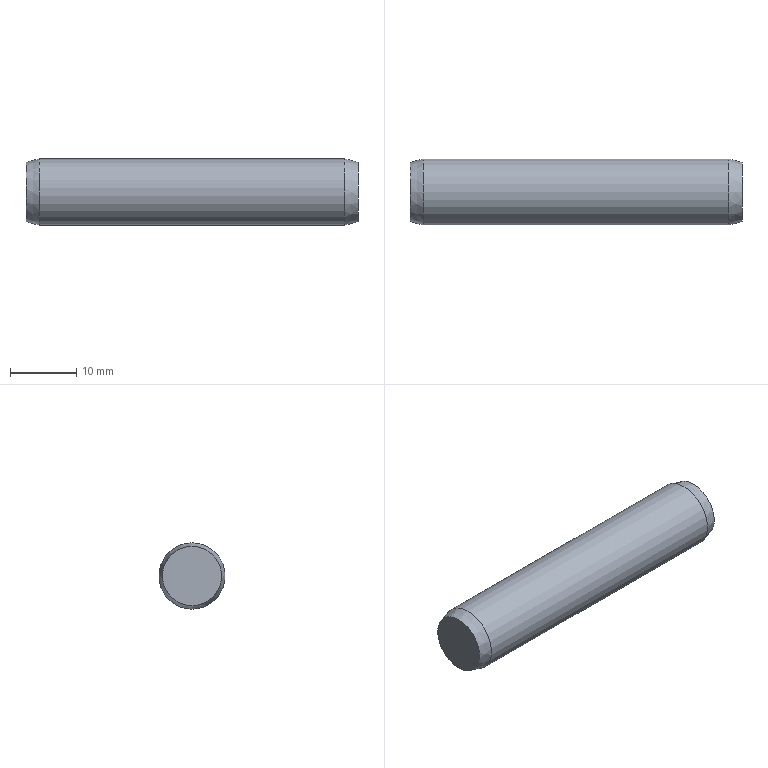Component | NX | GB-T119_1-2000_10X50 | 1 solid | 5 faces | box 50 x 10 x 10 mm | volume 3895 mm3 | plane 2 | cone 2 | cylinder 1 | commonest cylinder face diameters 10 x1
STEP:
#1=CARTESIAN_POINT('',(0.,0.,0.));
#2=DIRECTION('',(0.,0.,1.));
#3=DIRECTION('',(1.,0.,0.));
#4=AXIS2_PLACEMENT_3D('',#1,#2,#3);
#5=CARTESIAN_POINT('',(30.,-40.,-165.536));
#6=VERTEX_POINT('',#5);
#7=CARTESIAN_POINT('',(30.,-40.,-170.));
#8=DIRECTION('',(-1.,0.,0.));
#9=DIRECTION('',(0.,0.,1.));
#10=AXIS2_PLACEMENT_3D('',#7,#8,#9);
#11=CIRCLE('',#10,4.464);
#12=CARTESIAN_POINT('',(30.,-40.,-170.));
#13=DIRECTION('',(-1.,0.,0.));
#14=DIRECTION('',(0.,0.,1.));
#15=AXIS2_PLACEMENT_3D('',#12,#13,#14);
#16=PLANE('',#15);
#17=CARTESIAN_POINT('',(0.,0.));
#18=DIRECTION('',(1.,0.));
#19=AXIS2_PLACEMENT_2D('',#17,#18);
#20=CIRCLE('',#19,4.464);
#21=(GEOMETRIC_REPRESENTATION_CONTEXT(2)PARAMETRIC_REPRESENTATION_CONTEXT()REPRESENTATION_CONTEXT('',''));
#22=DEFINITIONAL_REPRESENTATION('',(#20),#21);
#23=PCURVE('',#16,#22);
#24=CARTESIAN_POINT('',(30.,-40.,-170.));
#25=DIRECTION('',(1.,0.,0.));
#26=DIRECTION('',(0.,0.,-1.));
#27=AXIS2_PLACEMENT_3D('',#24,#25,#26);
#28=CONICAL_SURFACE('',#27,4.464,0.2618);
#29=CARTESIAN_POINT('',(9.425,0.));
#30=DIRECTION('',(-1.,0.));
#31=VECTOR('',#30,1.);
#32=LINE('',#29,#31);
#33=(GEOMETRIC_REPRESENTATION_CONTEXT(2)PARAMETRIC_REPRESENTATION_CONTEXT()REPRESENTATION_CONTEXT('',''));
#34=DEFINITIONAL_REPRESENTATION('',(#32),#33);
#35=PCURVE('',#28,#34);
#36=SURFACE_CURVE('',#11,(#23,#35),.PCURVE_S1.);
#37=EDGE_CURVE('',#6,#6,#36,.T.);
#38=ORIENTED_EDGE('',*,*,#37,.T.);
#39=EDGE_LOOP('',(#38));
#40=FACE_BOUND('',#39,.T.);
#41=ADVANCED_FACE('',(#40),#16,.T.);
#42=CARTESIAN_POINT('',(32.,-40.,-165.));
#43=VERTEX_POINT('',#42);
#44=CARTESIAN_POINT('',(32.,-40.,-170.));
#45=DIRECTION('',(-1.,0.,0.));
#46=DIRECTION('',(0.,0.,1.));
#47=AXIS2_PLACEMENT_3D('',#44,#45,#46);
#48=CIRCLE('',#47,5.);
#49=CARTESIAN_POINT('',(9.425,2.));
#50=DIRECTION('',(-1.,0.));
#51=VECTOR('',#50,1.);
#52=LINE('',#49,#51);
#53=(GEOMETRIC_REPRESENTATION_CONTEXT(2)PARAMETRIC_REPRESENTATION_CONTEXT()REPRESENTATION_CONTEXT('',''));
#54=DEFINITIONAL_REPRESENTATION('',(#52),#53);
#55=PCURVE('',#28,#54);
#56=CARTESIAN_POINT('',(80.,-40.,-170.));
#57=DIRECTION('',(-1.,0.,0.));
#58=DIRECTION('',(0.,0.,1.));
#59=AXIS2_PLACEMENT_3D('',#56,#57,#58);
#60=CYLINDRICAL_SURFACE('',#59,5.);
#61=CARTESIAN_POINT('',(0.,48.));
#62=DIRECTION('',(1.,0.));
#63=VECTOR('',#62,1.);
#64=LINE('',#61,#63);
#65=(GEOMETRIC_REPRESENTATION_CONTEXT(2)PARAMETRIC_REPRESENTATION_CONTEXT()REPRESENTATION_CONTEXT('',''));
#66=DEFINITIONAL_REPRESENTATION('',(#64),#65);
#67=PCURVE('',#60,#66);
#68=SURFACE_CURVE('',#48,(#55,#67),.PCURVE_S1.);
#69=EDGE_CURVE('',#43,#43,#68,.T.);
#70=ORIENTED_EDGE('',*,*,#69,.T.);
#71=CARTESIAN_POINT('',(30.,-40.,-165.536));
#72=CARTESIAN_POINT('',(32.,-40.,-165.));
#73=B_SPLINE_CURVE_WITH_KNOTS('',1,(#71,#72),.UNSPECIFIED.,.F.,.F.,(2,2),(0.,2.071),.PIECEWISE_BEZIER_KNOTS.);
#74=CARTESIAN_POINT('',(3.142,0.));
#75=DIRECTION('',(0.,1.));
#76=VECTOR('',#75,1.);
#77=LINE('',#74,#76);
#78=(GEOMETRIC_REPRESENTATION_CONTEXT(2)PARAMETRIC_REPRESENTATION_CONTEXT()REPRESENTATION_CONTEXT('',''));
#79=DEFINITIONAL_REPRESENTATION('',(#77),#78);
#80=PCURVE('',#28,#79);
#81=CARTESIAN_POINT('',(9.425,0.));
#82=DIRECTION('',(0.,1.));
#83=VECTOR('',#82,1.);
#84=LINE('',#81,#83);
#85=(GEOMETRIC_REPRESENTATION_CONTEXT(2)PARAMETRIC_REPRESENTATION_CONTEXT()REPRESENTATION_CONTEXT('',''));
#86=DEFINITIONAL_REPRESENTATION('',(#84),#85);
#87=PCURVE('',#28,#86);
#88=SEAM_CURVE('',#73,(#80,#87),.PCURVE_S1.);
#89=EDGE_CURVE('',#6,#43,#88,.T.);
#90=ORIENTED_EDGE('',*,*,#89,.F.);
#91=ORIENTED_EDGE('',*,*,#37,.F.);
#92=ORIENTED_EDGE('',*,*,#89,.T.);
#93=EDGE_LOOP('',(#70,#90,#91,#92));
#94=FACE_BOUND('',#93,.T.);
#95=ADVANCED_FACE('',(#94),#28,.T.);
#96=CARTESIAN_POINT('',(78.,-40.,-165.));
#97=VERTEX_POINT('',#96);
#98=CARTESIAN_POINT('',(78.,-40.,-170.));
#99=DIRECTION('',(-1.,0.,0.));
#100=DIRECTION('',(0.,0.,1.));
#101=AXIS2_PLACEMENT_3D('',#98,#99,#100);
#102=CIRCLE('',#101,5.);
#103=CARTESIAN_POINT('',(0.,2.));
#104=DIRECTION('',(1.,0.));
#105=VECTOR('',#104,1.);
#106=LINE('',#103,#105);
#107=(GEOMETRIC_REPRESENTATION_CONTEXT(2)PARAMETRIC_REPRESENTATION_CONTEXT()REPRESENTATION_CONTEXT('',''));
#108=DEFINITIONAL_REPRESENTATION('',(#106),#107);
#109=PCURVE('',#60,#108);
#110=CARTESIAN_POINT('',(78.,-40.,-170.));
#111=DIRECTION('',(-1.,0.,0.));
#112=DIRECTION('',(0.,0.,1.));
#113=AXIS2_PLACEMENT_3D('',#110,#111,#112);
#114=CONICAL_SURFACE('',#113,5.,0.2618);
#115=CARTESIAN_POINT('',(0.,0.));
#116=DIRECTION('',(1.,0.));
#117=VECTOR('',#116,1.);
#118=LINE('',#115,#117);
#119=(GEOMETRIC_REPRESENTATION_CONTEXT(2)PARAMETRIC_REPRESENTATION_CONTEXT()REPRESENTATION_CONTEXT('',''));
#120=DEFINITIONAL_REPRESENTATION('',(#118),#119);
#121=PCURVE('',#114,#120);
#122=SURFACE_CURVE('',#102,(#109,#121),.PCURVE_S1.);
#123=EDGE_CURVE('',#97,#97,#122,.T.);
#124=ORIENTED_EDGE('',*,*,#123,.T.);
#125=CARTESIAN_POINT('',(78.,-40.,-165.));
#126=CARTESIAN_POINT('',(32.,-40.,-165.));
#127=B_SPLINE_CURVE_WITH_KNOTS('',1,(#125,#126),.UNSPECIFIED.,.F.,.F.,(2,2),(2.,48.),.PIECEWISE_BEZIER_KNOTS.);
#128=CARTESIAN_POINT('',(6.283,0.));
#129=DIRECTION('',(0.,1.));
#130=VECTOR('',#129,1.);
#131=LINE('',#128,#130);
#132=(GEOMETRIC_REPRESENTATION_CONTEXT(2)PARAMETRIC_REPRESENTATION_CONTEXT()REPRESENTATION_CONTEXT('',''));
#133=DEFINITIONAL_REPRESENTATION('',(#131),#132);
#134=PCURVE('',#60,#133);
#135=CARTESIAN_POINT('',(0.,0.));
#136=DIRECTION('',(0.,1.));
#137=VECTOR('',#136,1.);
#138=LINE('',#135,#137);
#139=(GEOMETRIC_REPRESENTATION_CONTEXT(2)PARAMETRIC_REPRESENTATION_CONTEXT()REPRESENTATION_CONTEXT('',''));
#140=DEFINITIONAL_REPRESENTATION('',(#138),#139);
#141=PCURVE('',#60,#140);
#142=SEAM_CURVE('',#127,(#134,#141),.PCURVE_S1.);
#143=EDGE_CURVE('',#97,#43,#142,.T.);
#144=ORIENTED_EDGE('',*,*,#143,.T.);
#145=ORIENTED_EDGE('',*,*,#69,.F.);
#146=ORIENTED_EDGE('',*,*,#143,.F.);
#147=EDGE_LOOP('',(#124,#144,#145,#146));
#148=FACE_BOUND('',#147,.T.);
#149=ADVANCED_FACE('',(#148),#60,.T.);
#150=CARTESIAN_POINT('',(80.,-40.,-165.536));
#151=VERTEX_POINT('',#150);
#152=CARTESIAN_POINT('',(80.,-40.,-170.));
#153=DIRECTION('',(-1.,0.,0.));
#154=DIRECTION('',(0.,0.,1.));
#155=AXIS2_PLACEMENT_3D('',#152,#153,#154);
#156=CIRCLE('',#155,4.464);
#157=CARTESIAN_POINT('',(0.,-2.));
#158=DIRECTION('',(1.,0.));
#159=VECTOR('',#158,1.);
#160=LINE('',#157,#159);
#161=(GEOMETRIC_REPRESENTATION_CONTEXT(2)PARAMETRIC_REPRESENTATION_CONTEXT()REPRESENTATION_CONTEXT('',''));
#162=DEFINITIONAL_REPRESENTATION('',(#160),#161);
#163=PCURVE('',#114,#162);
#164=CARTESIAN_POINT('',(80.,-40.,-174.464));
#165=DIRECTION('',(1.,0.,0.));
#166=DIRECTION('',(0.,0.,-1.));
#167=AXIS2_PLACEMENT_3D('',#164,#165,#166);
#168=PLANE('',#167);
#169=CARTESIAN_POINT('',(-8.928,0.));
#170=CARTESIAN_POINT('',(-8.928,7.732));
#171=CARTESIAN_POINT('',(-2.232,3.866));
#172=CARTESIAN_POINT('',(4.464,0.));
#173=CARTESIAN_POINT('',(-2.232,-3.866));
#174=CARTESIAN_POINT('',(-8.928,-7.732));
#175=CARTESIAN_POINT('',(-8.928,0.));
#176=(BOUNDED_CURVE()B_SPLINE_CURVE(2,(#169,#170,#171,#172,#173,#174,#175),.UNSPECIFIED.,.T.,.F.)B_SPLINE_CURVE_WITH_KNOTS((1,2,2,2,2,1),(-2.094,0.,2.094,4.189,6.283,8.378),.UNSPECIFIED.)CURVE()GEOMETRIC_REPRESENTATION_ITEM()RATIONAL_B_SPLINE_CURVE((1.,0.5,1.,0.5,1.,0.5,1.))REPRESENTATION_ITEM(''));
#177=(GEOMETRIC_REPRESENTATION_CONTEXT(2)PARAMETRIC_REPRESENTATION_CONTEXT()REPRESENTATION_CONTEXT('',''));
#178=DEFINITIONAL_REPRESENTATION('',(#176),#177);
#179=PCURVE('',#168,#178);
#180=SURFACE_CURVE('',#156,(#163,#179),.PCURVE_S1.);
#181=EDGE_CURVE('',#151,#151,#180,.T.);
#182=ORIENTED_EDGE('',*,*,#181,.T.);
#183=CARTESIAN_POINT('',(80.,-40.,-165.536));
#184=CARTESIAN_POINT('',(78.,-40.,-165.));
#185=B_SPLINE_CURVE_WITH_KNOTS('',1,(#183,#184),.UNSPECIFIED.,.F.,.F.,(2,2),(-2.071,0.),.PIECEWISE_BEZIER_KNOTS.);
#186=CARTESIAN_POINT('',(6.283,0.));
#187=DIRECTION('',(0.,1.));
#188=VECTOR('',#187,1.);
#189=LINE('',#186,#188);
#190=(GEOMETRIC_REPRESENTATION_CONTEXT(2)PARAMETRIC_REPRESENTATION_CONTEXT()REPRESENTATION_CONTEXT('',''));
#191=DEFINITIONAL_REPRESENTATION('',(#189),#190);
#192=PCURVE('',#114,#191);
#193=CARTESIAN_POINT('',(0.,0.));
#194=DIRECTION('',(0.,1.));
#195=VECTOR('',#194,1.);
#196=LINE('',#193,#195);
#197=(GEOMETRIC_REPRESENTATION_CONTEXT(2)PARAMETRIC_REPRESENTATION_CONTEXT()REPRESENTATION_CONTEXT('',''));
#198=DEFINITIONAL_REPRESENTATION('',(#196),#197);
#199=PCURVE('',#114,#198);
#200=SEAM_CURVE('',#185,(#192,#199),.PCURVE_S1.);
#201=EDGE_CURVE('',#151,#97,#200,.T.);
#202=ORIENTED_EDGE('',*,*,#201,.T.);
#203=ORIENTED_EDGE('',*,*,#123,.F.);
#204=ORIENTED_EDGE('',*,*,#201,.F.);
#205=EDGE_LOOP('',(#182,#202,#203,#204));
#206=FACE_BOUND('',#205,.T.);
#207=ADVANCED_FACE('',(#206),#114,.T.);
#208=ORIENTED_EDGE('',*,*,#181,.F.);
#209=EDGE_LOOP('',(#208));
#210=FACE_BOUND('',#209,.T.);
#211=ADVANCED_FACE('',(#210),#168,.T.);
#212=CLOSED_SHELL('',(#41,#95,#149,#207,#211));
#213=MANIFOLD_SOLID_BREP('',#212);
#214=(LENGTH_UNIT()NAMED_UNIT(*)SI_UNIT(.MILLI.,.METRE.));
#215=UNCERTAINTY_MEASURE_WITH_UNIT(LENGTH_MEASURE(0.00001),#214,'','');
#216=(NAMED_UNIT(*)PLANE_ANGLE_UNIT()SI_UNIT($,.RADIAN.));
#217=(NAMED_UNIT(*)SI_UNIT($,.STERADIAN.)SOLID_ANGLE_UNIT());
#218=(GEOMETRIC_REPRESENTATION_CONTEXT(3)GLOBAL_UNCERTAINTY_ASSIGNED_CONTEXT((#215))GLOBAL_UNIT_ASSIGNED_CONTEXT((#214,#216,#217))REPRESENTATION_CONTEXT('',''));
#219=ADVANCED_BREP_SHAPE_REPRESENTATION('',(#4,#213),#218);